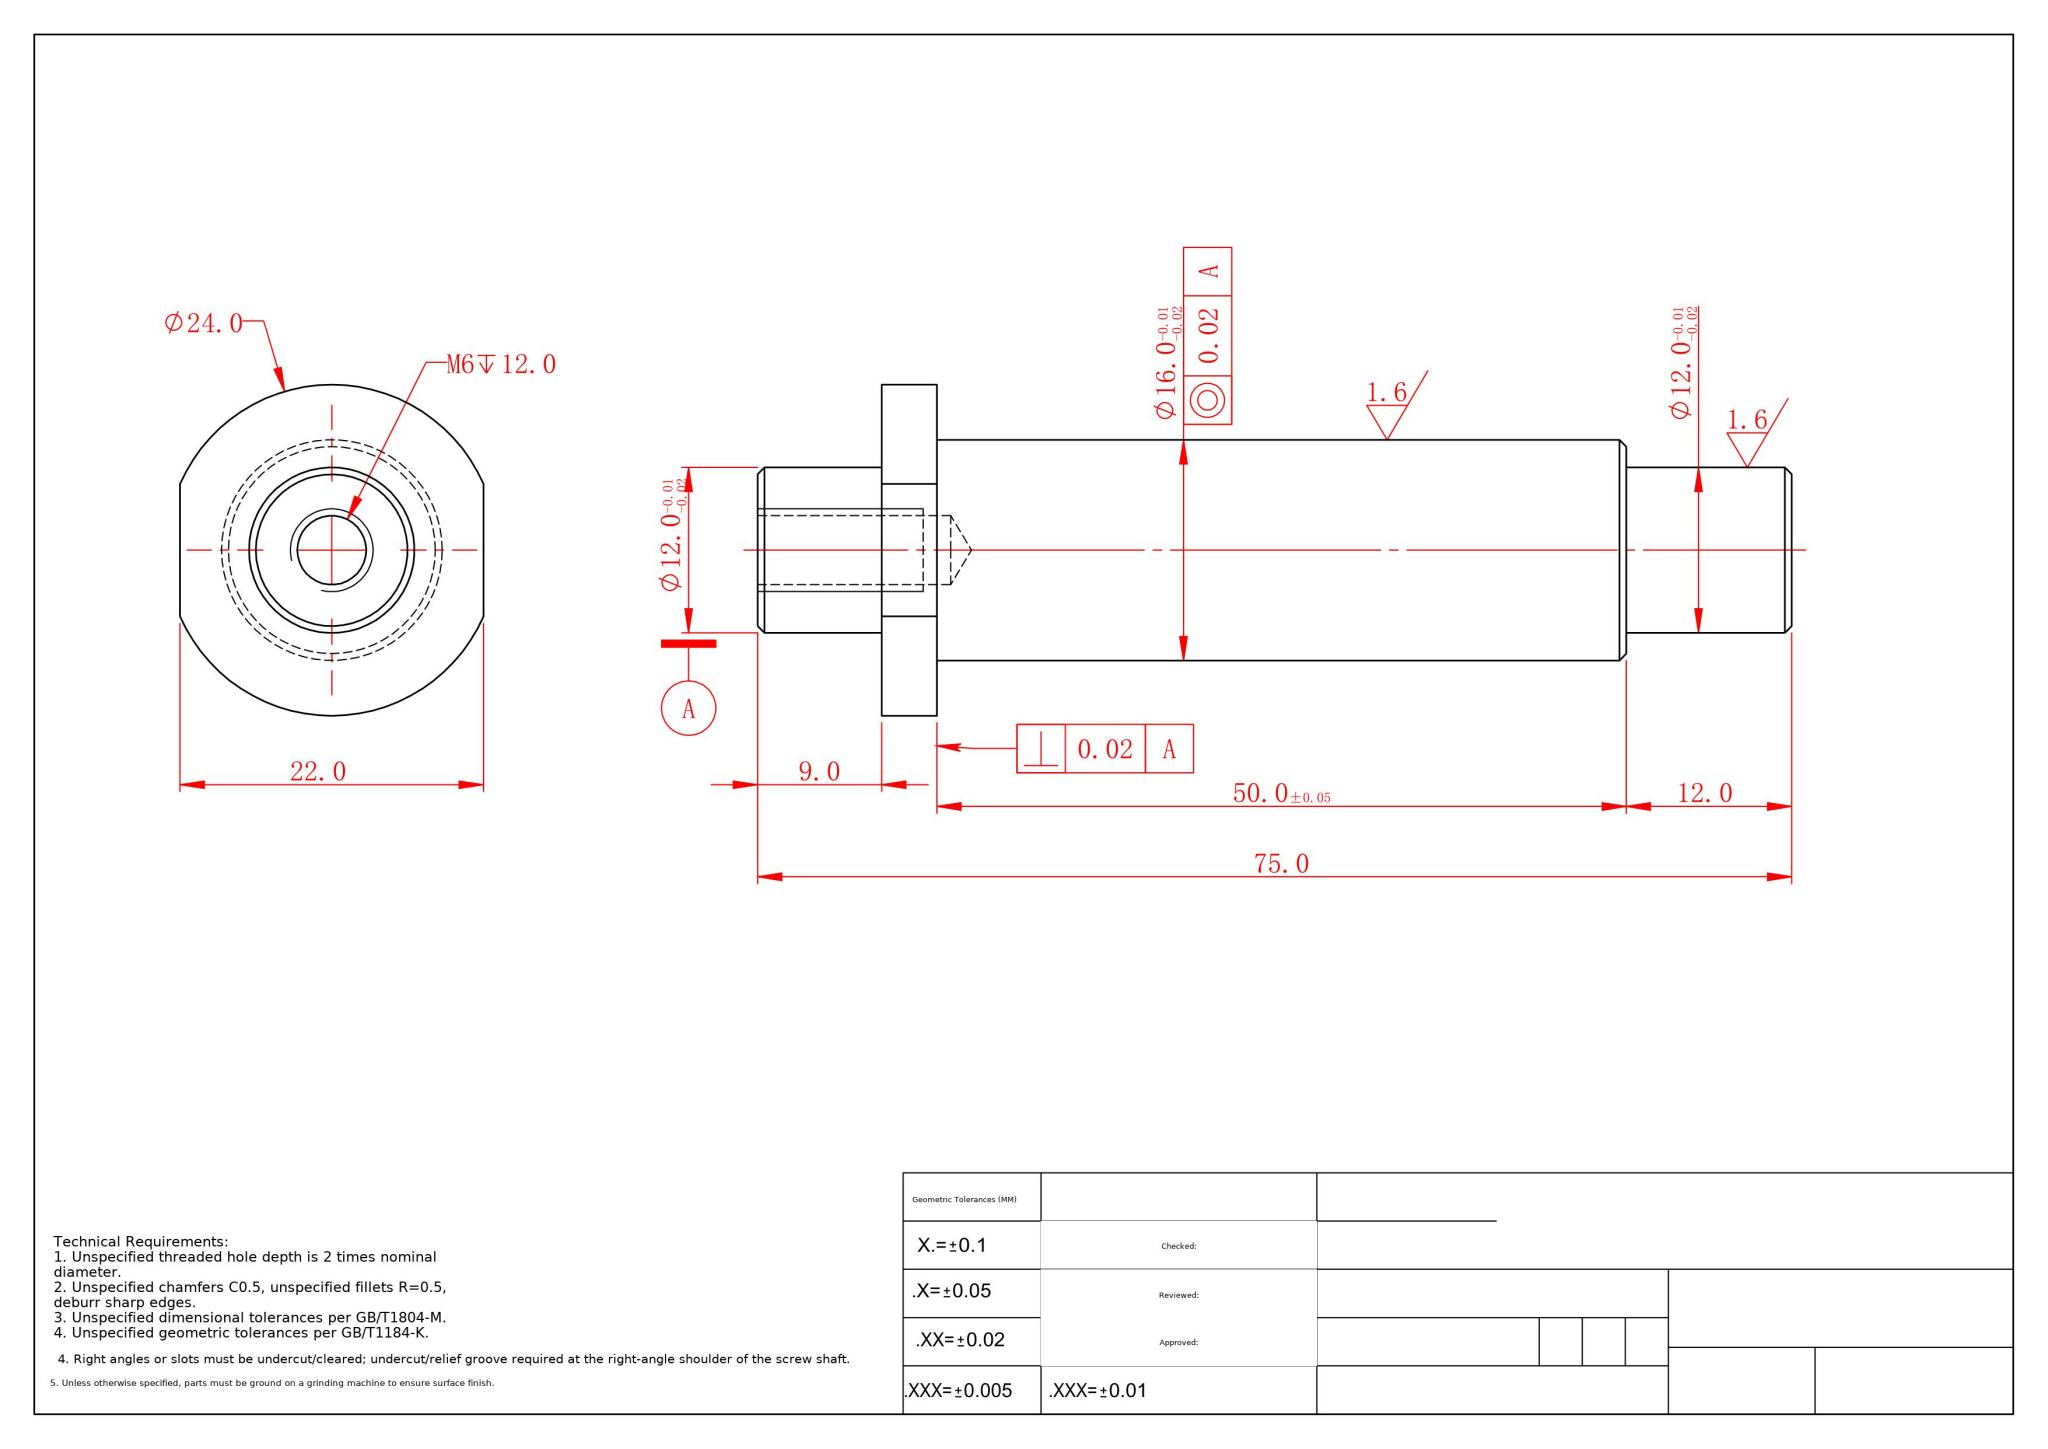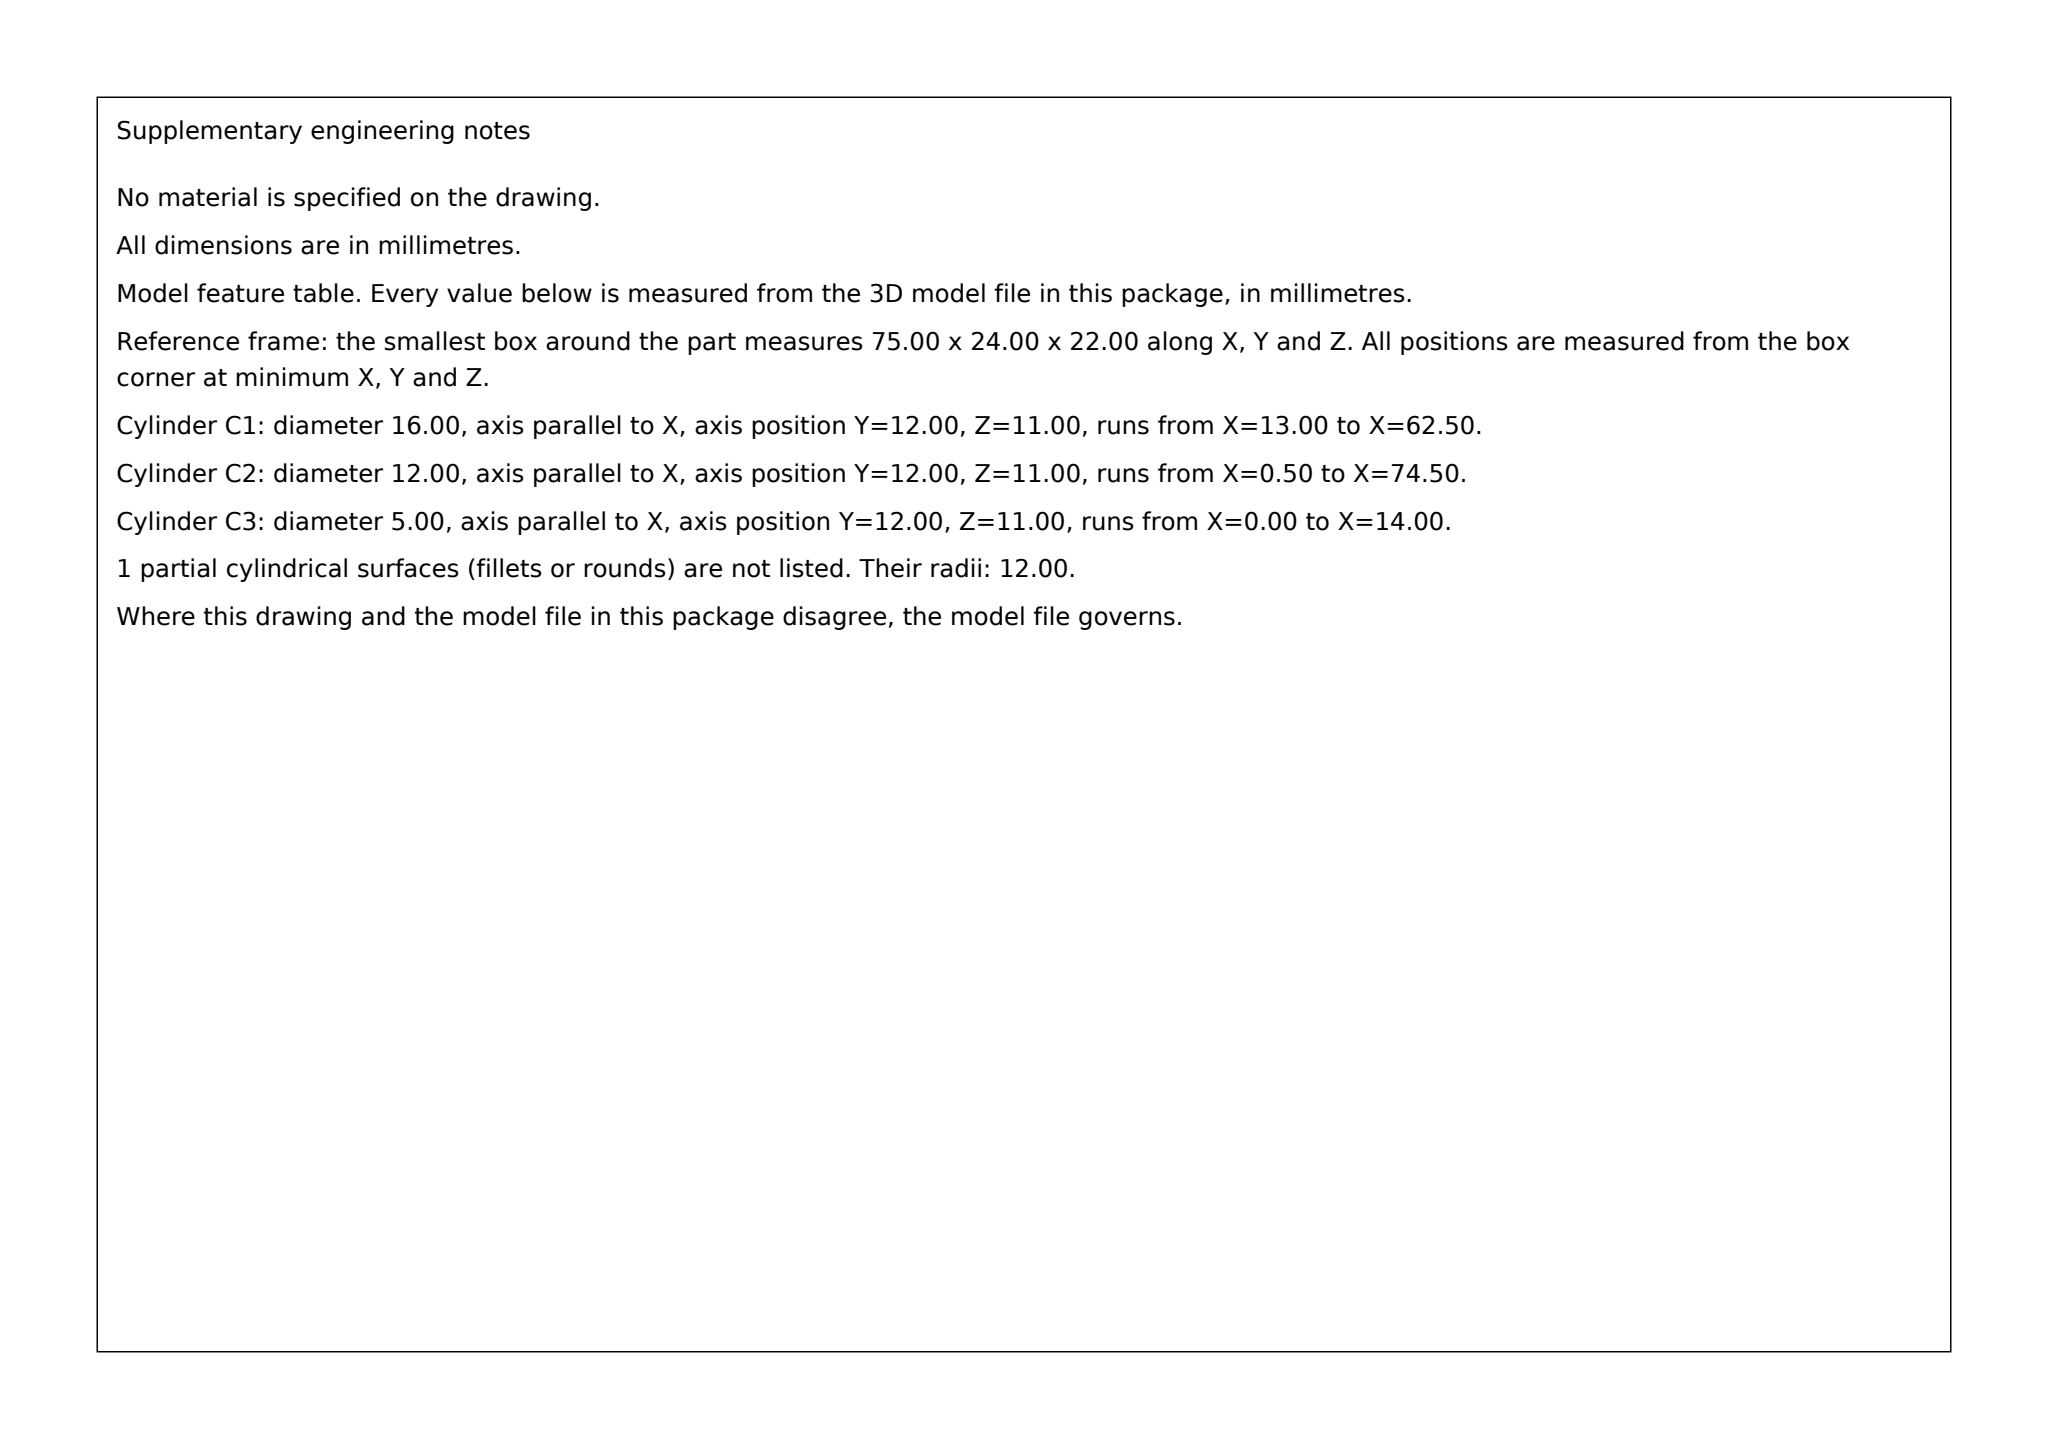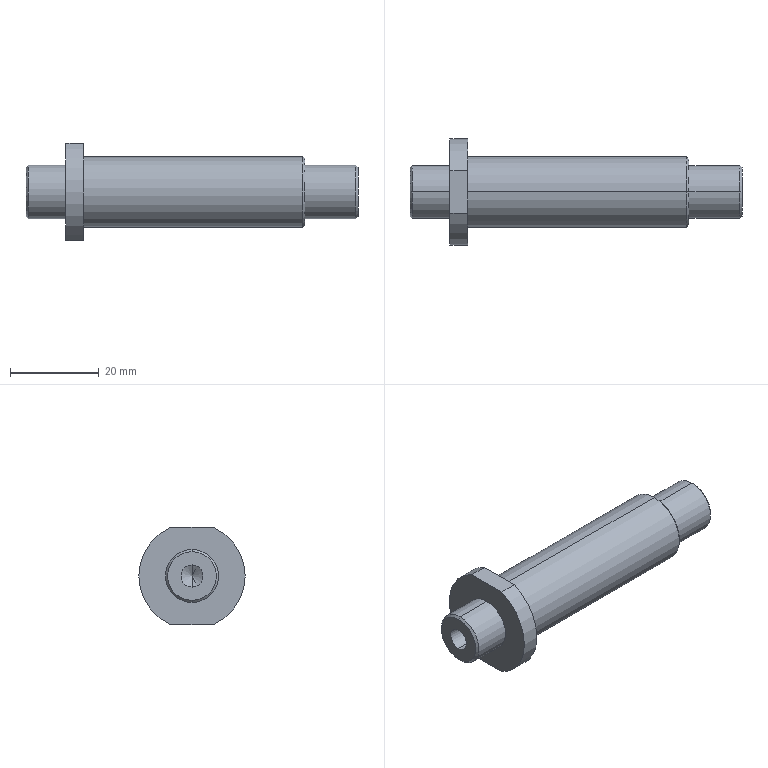Part | SolidWorks | mm | 1 solid | 25 faces | box 75 x 24 x 22 mm | volume 13886 mm3 | cylinder 10 | cone 8 | plane 7 | commonest cylinder face diameters 12 x4 5 x2 16 x2 24 x2
build123d program:
from build123d import *

# Parameters (mm, degrees)
M6_TAPPED_HOLE1_D     = 5
M6_TAPPED_HOLE1_DEPTH = 14
M6_TAPPED_HOLE1_TIP   = 1.502
CUT_EXTRUDE1_REACH    = 66.281
SKETCH4_W             = 1.714
SKETCH4_H             = 24.788
CHAMFER1_SIZE         = 0.5


with BuildPart() as part:
    # Sketch1 → Revolve1 (revolve)
    with BuildSketch(Plane.XY, mode=Mode.PRIVATE) as revolve1_sk:
        Polygon((-37.5, 0), (37.5, 0), (37.5, 6), (25.5, 6), (25.5, 8), (-24.5, 8), (-24.5, 12), (-28.5, 12), (-28.5, 6), (-37.5, 6), align=None)
    revolve(revolve1_sk.sketch.rotate(Axis((0, 0, 0), (1, 0, 0)), 90), axis=Axis((0, 0, 0), (1, 0, 0)))

    # M6 Tapped Hole1
    with Locations(Plane.ZY.offset(37.5)):
        with Locations((0, 0)):
            Hole(M6_TAPPED_HOLE1_D / 2, depth=M6_TAPPED_HOLE1_DEPTH)
            with Locations((0, 0, -(M6_TAPPED_HOLE1_DEPTH + M6_TAPPED_HOLE1_TIP / 2))):  # 118° drill point
                Cone(0, M6_TAPPED_HOLE1_D / 2, M6_TAPPED_HOLE1_TIP, mode=Mode.SUBTRACT)

    # Sketch4 → Cut-Extrude1 (cut, up to next)
    with BuildSketch(Plane(origin=(-24.5, 0, 0), x_dir=(0, 0, -1), z_dir=(1, 0, 0)), mode=Mode.PRIVATE) as cut_extrude1_sk1:
        with Locations((-11.857, 1.847)):
            Rectangle(SKETCH4_W, SKETCH4_H)
    cut_extrude1_tool1 = extrude(cut_extrude1_sk1.sketch, amount=-CUT_EXTRUDE1_REACH, mode=Mode.PRIVATE) & part.part
    # Sketch4 → Cut-Extrude1 (cut, up to next)
    with BuildSketch(Plane(origin=(-24.5, 0, 0), x_dir=(0, 0, -1), z_dir=(1, 0, 0)), mode=Mode.PRIVATE) as cut_extrude1_sk2:
        with Locations((11.857, 1.847)):
            Rectangle(SKETCH4_W, SKETCH4_H)
    cut_extrude1_tool2 = extrude(cut_extrude1_sk2.sketch, amount=-CUT_EXTRUDE1_REACH, mode=Mode.PRIVATE) & part.part
    add(cut_extrude1_tool1.solids().sort_by_distance((-24.5, 1.847, 11.857))[0], mode=Mode.SUBTRACT)
    add(cut_extrude1_tool2.solids().sort_by_distance((-24.5, 1.847, -11.857))[0], mode=Mode.SUBTRACT)

    # Chamfer1
    chamfer1_edges = [part.edges().sort_by_distance(p)[0] for p in [
        (25.5, 0, -8),
        (37.5, 0, -6),
        (-37.5, 0, -6),
    ]]
    chamfer(chamfer1_edges, length=CHAMFER1_SIZE)


solid = part.part
STEP:
#1=CARTESIAN_POINT('',(37.5,0.,-5.5));
#2=VERTEX_POINT('',#1);
#3=CARTESIAN_POINT('',(37.5,0.,5.5));
#4=VERTEX_POINT('',#3);
#5=CARTESIAN_POINT('',(37.5,0.,0.));
#6=DIRECTION('',(1.,0.,0.));
#7=DIRECTION('',(0.,0.,1.));
#8=AXIS2_PLACEMENT_3D('',#5,#6,#7);
#9=CIRCLE('',#8,5.5);
#10=EDGE_CURVE('',#2,#4,#9,.T.);
#11=ORIENTED_EDGE('',*,*,#10,.F.);
#12=CARTESIAN_POINT('',(37.,0.,-6.));
#13=VERTEX_POINT('',#12);
#14=CARTESIAN_POINT('',(37.,0.,-6.));
#15=DIRECTION('',(-0.7071,0.,-0.7071));
#16=VECTOR('',#15,1000.);
#17=LINE('',#14,#16);
#18=EDGE_CURVE('',#2,#13,#17,.T.);
#19=ORIENTED_EDGE('',*,*,#18,.T.);
#20=CARTESIAN_POINT('',(37.,0.,6.));
#21=VERTEX_POINT('',#20);
#22=CARTESIAN_POINT('',(37.,0.,0.));
#23=DIRECTION('',(-1.,0.,0.));
#24=DIRECTION('',(0.,0.,1.));
#25=AXIS2_PLACEMENT_3D('',#22,#23,#24);
#26=CIRCLE('',#25,6.);
#27=EDGE_CURVE('',#21,#13,#26,.T.);
#28=ORIENTED_EDGE('',*,*,#27,.F.);
#29=CARTESIAN_POINT('',(37.,0.,6.));
#30=DIRECTION('',(-0.7071,0.,0.7071));
#31=VECTOR('',#30,1000.);
#32=LINE('',#29,#31);
#33=EDGE_CURVE('',#4,#21,#32,.T.);
#34=ORIENTED_EDGE('',*,*,#33,.F.);
#35=EDGE_LOOP('',(#11,#19,#28,#34));
#36=FACE_OUTER_BOUND('',#35,.T.);
#37=CARTESIAN_POINT('',(37.,0.,0.));
#38=DIRECTION('',(-1.,0.,0.));
#39=DIRECTION('',(0.,0.,1.));
#40=AXIS2_PLACEMENT_3D('',#37,#38,#39);
#41=CONICAL_SURFACE('',#40,6.,0.7854);
#42=ADVANCED_FACE('',(#36),#41,.T.);
#43=CARTESIAN_POINT('',(25.5,0.,-7.5));
#44=VERTEX_POINT('',#43);
#45=CARTESIAN_POINT('',(25.5,0.,7.5));
#46=VERTEX_POINT('',#45);
#47=CARTESIAN_POINT('',(25.5,0.,0.));
#48=DIRECTION('',(1.,0.,0.));
#49=DIRECTION('',(0.,0.,1.));
#50=AXIS2_PLACEMENT_3D('',#47,#48,#49);
#51=CIRCLE('',#50,7.5);
#52=EDGE_CURVE('',#44,#46,#51,.T.);
#53=ORIENTED_EDGE('',*,*,#52,.F.);
#54=CARTESIAN_POINT('',(25.,0.,-8.));
#55=VERTEX_POINT('',#54);
#56=CARTESIAN_POINT('',(25.,0.,-8.));
#57=DIRECTION('',(-0.7071,0.,-0.7071));
#58=VECTOR('',#57,1000.);
#59=LINE('',#56,#58);
#60=EDGE_CURVE('',#44,#55,#59,.T.);
#61=ORIENTED_EDGE('',*,*,#60,.T.);
#62=CARTESIAN_POINT('',(25.,0.,8.));
#63=VERTEX_POINT('',#62);
#64=CARTESIAN_POINT('',(25.,0.,0.));
#65=DIRECTION('',(-1.,0.,0.));
#66=DIRECTION('',(0.,0.,1.));
#67=AXIS2_PLACEMENT_3D('',#64,#65,#66);
#68=CIRCLE('',#67,8.);
#69=EDGE_CURVE('',#63,#55,#68,.T.);
#70=ORIENTED_EDGE('',*,*,#69,.F.);
#71=CARTESIAN_POINT('',(25.,0.,8.));
#72=DIRECTION('',(-0.7071,0.,0.7071));
#73=VECTOR('',#72,1000.);
#74=LINE('',#71,#73);
#75=EDGE_CURVE('',#46,#63,#74,.T.);
#76=ORIENTED_EDGE('',*,*,#75,.F.);
#77=EDGE_LOOP('',(#53,#61,#70,#76));
#78=FACE_OUTER_BOUND('',#77,.T.);
#79=CARTESIAN_POINT('',(25.,0.,0.));
#80=DIRECTION('',(-1.,0.,0.));
#81=DIRECTION('',(0.,0.,1.));
#82=AXIS2_PLACEMENT_3D('',#79,#80,#81);
#83=CONICAL_SURFACE('',#82,8.,0.7854);
#84=ADVANCED_FACE('',(#78),#83,.T.);
#85=CARTESIAN_POINT('',(-37.5,0.,5.5));
#86=VERTEX_POINT('',#85);
#87=CARTESIAN_POINT('',(-37.5,0.,-5.5));
#88=VERTEX_POINT('',#87);
#89=CARTESIAN_POINT('',(-37.5,0.,0.));
#90=DIRECTION('',(-1.,0.,0.));
#91=DIRECTION('',(0.,0.,-1.));
#92=AXIS2_PLACEMENT_3D('',#89,#90,#91);
#93=CIRCLE('',#92,5.5);
#94=EDGE_CURVE('',#86,#88,#93,.T.);
#95=ORIENTED_EDGE('',*,*,#94,.F.);
#96=CARTESIAN_POINT('',(-37.,0.,6.));
#97=VERTEX_POINT('',#96);
#98=CARTESIAN_POINT('',(-37.5,0.,5.5));
#99=DIRECTION('',(0.7071,0.,0.7071));
#100=VECTOR('',#99,1000.);
#101=LINE('',#98,#100);
#102=EDGE_CURVE('',#86,#97,#101,.T.);
#103=ORIENTED_EDGE('',*,*,#102,.T.);
#104=CARTESIAN_POINT('',(-37.,0.,-6.));
#105=VERTEX_POINT('',#104);
#106=CARTESIAN_POINT('',(-37.,0.,0.));
#107=DIRECTION('',(1.,0.,0.));
#108=DIRECTION('',(0.,0.,-1.));
#109=AXIS2_PLACEMENT_3D('',#106,#107,#108);
#110=CIRCLE('',#109,6.);
#111=EDGE_CURVE('',#105,#97,#110,.T.);
#112=ORIENTED_EDGE('',*,*,#111,.F.);
#113=CARTESIAN_POINT('',(-37.5,0.,-5.5));
#114=DIRECTION('',(0.7071,0.,-0.7071));
#115=VECTOR('',#114,1000.);
#116=LINE('',#113,#115);
#117=EDGE_CURVE('',#88,#105,#116,.T.);
#118=ORIENTED_EDGE('',*,*,#117,.F.);
#119=EDGE_LOOP('',(#95,#103,#112,#118));
#120=FACE_OUTER_BOUND('',#119,.T.);
#121=CARTESIAN_POINT('',(-37.5,0.,0.));
#122=DIRECTION('',(1.,0.,0.));
#123=DIRECTION('',(0.,0.,-1.));
#124=AXIS2_PLACEMENT_3D('',#121,#122,#123);
#125=CONICAL_SURFACE('',#124,5.5,0.7854);
#126=ADVANCED_FACE('',(#120),#125,.T.);
#127=CARTESIAN_POINT('',(-23.5,0.,-2.5));
#128=VERTEX_POINT('',#127);
#129=CARTESIAN_POINT('',(-23.5,0.,2.5));
#130=VERTEX_POINT('',#129);
#131=CARTESIAN_POINT('',(-23.5,0.,0.));
#132=DIRECTION('',(-1.,0.,0.));
#133=DIRECTION('',(0.,0.,1.));
#134=AXIS2_PLACEMENT_3D('',#131,#132,#133);
#135=CIRCLE('',#134,2.5);
#136=EDGE_CURVE('',#128,#130,#135,.T.);
#137=ORIENTED_EDGE('',*,*,#136,.F.);
#138=CARTESIAN_POINT('',(-37.5,0.,-2.5));
#139=VERTEX_POINT('',#138);
#140=CARTESIAN_POINT('',(-37.5,0.,-2.5));
#141=DIRECTION('',(-1.,0.,0.));
#142=VECTOR('',#141,1000.);
#143=LINE('',#140,#142);
#144=EDGE_CURVE('',#128,#139,#143,.T.);
#145=ORIENTED_EDGE('',*,*,#144,.T.);
#146=CARTESIAN_POINT('',(-37.5,0.,2.5));
#147=VERTEX_POINT('',#146);
#148=CARTESIAN_POINT('',(-37.5,0.,0.));
#149=DIRECTION('',(-1.,0.,0.));
#150=DIRECTION('',(0.,0.,1.));
#151=AXIS2_PLACEMENT_3D('',#148,#149,#150);
#152=CIRCLE('',#151,2.5);
#153=EDGE_CURVE('',#139,#147,#152,.T.);
#154=ORIENTED_EDGE('',*,*,#153,.T.);
#155=CARTESIAN_POINT('',(-37.5,0.,2.5));
#156=DIRECTION('',(-1.,0.,0.));
#157=VECTOR('',#156,1000.);
#158=LINE('',#155,#157);
#159=EDGE_CURVE('',#130,#147,#158,.T.);
#160=ORIENTED_EDGE('',*,*,#159,.F.);
#161=EDGE_LOOP('',(#137,#145,#154,#160));
#162=FACE_OUTER_BOUND('',#161,.T.);
#163=CARTESIAN_POINT('',(-37.5,0.,0.));
#164=DIRECTION('',(-1.,0.,0.));
#165=DIRECTION('',(0.,0.,1.));
#166=AXIS2_PLACEMENT_3D('',#163,#164,#165);
#167=CYLINDRICAL_SURFACE('',#166,2.5);
#168=ADVANCED_FACE('',(#162),#167,.F.);
#169=CARTESIAN_POINT('',(-21.998,-0.,0.));
#170=VERTEX_POINT('',#169);
#171=CARTESIAN_POINT('',(-23.5,0.,2.5));
#172=DIRECTION('',(-0.515,0.,0.8572));
#173=VECTOR('',#172,1000.);
#174=LINE('',#171,#173);
#175=EDGE_CURVE('',#170,#130,#174,.T.);
#176=ORIENTED_EDGE('',*,*,#175,.F.);
#177=CARTESIAN_POINT('',(-23.5,0.,-2.5));
#178=DIRECTION('',(-0.515,0.,-0.8572));
#179=VECTOR('',#178,1000.);
#180=LINE('',#177,#179);
#181=EDGE_CURVE('',#170,#128,#180,.T.);
#182=ORIENTED_EDGE('',*,*,#181,.T.);
#183=ORIENTED_EDGE('',*,*,#136,.T.);
#184=EDGE_LOOP('',(#176,#182,#183));
#185=FACE_OUTER_BOUND('',#184,.T.);
#186=CARTESIAN_POINT('',(-23.5,0.,0.));
#187=DIRECTION('',(-1.,0.,0.));
#188=DIRECTION('',(0.,0.,1.));
#189=AXIS2_PLACEMENT_3D('',#186,#187,#188);
#190=CONICAL_SURFACE('',#189,2.5,1.03);
#191=ADVANCED_FACE('',(#185),#190,.F.);
#192=CARTESIAN_POINT('',(-28.5,0.,6.));
#193=VERTEX_POINT('',#192);
#194=CARTESIAN_POINT('',(-28.5,0.,-6.));
#195=VERTEX_POINT('',#194);
#196=CARTESIAN_POINT('',(-28.5,0.,0.));
#197=DIRECTION('',(-1.,0.,0.));
#198=DIRECTION('',(0.,0.,1.));
#199=AXIS2_PLACEMENT_3D('',#196,#197,#198);
#200=CIRCLE('',#199,6.);
#201=EDGE_CURVE('',#193,#195,#200,.T.);
#202=ORIENTED_EDGE('',*,*,#201,.T.);
#203=CARTESIAN_POINT('',(0.,0.,-6.));
#204=DIRECTION('',(-1.,0.,0.));
#205=VECTOR('',#204,1000.);
#206=LINE('',#203,#205);
#207=EDGE_CURVE('',#195,#105,#206,.T.);
#208=ORIENTED_EDGE('',*,*,#207,.T.);
#209=ORIENTED_EDGE('',*,*,#111,.T.);
#210=CARTESIAN_POINT('',(0.,0.,6.));
#211=DIRECTION('',(-1.,0.,0.));
#212=VECTOR('',#211,1000.);
#213=LINE('',#210,#212);
#214=EDGE_CURVE('',#193,#97,#213,.T.);
#215=ORIENTED_EDGE('',*,*,#214,.F.);
#216=EDGE_LOOP('',(#202,#208,#209,#215));
#217=FACE_OUTER_BOUND('',#216,.T.);
#218=CARTESIAN_POINT('',(0.,0.,0.));
#219=DIRECTION('',(-1.,0.,0.));
#220=DIRECTION('',(0.,0.,1.));
#221=AXIS2_PLACEMENT_3D('',#218,#219,#220);
#222=CYLINDRICAL_SURFACE('',#221,6.);
#223=ADVANCED_FACE('',(#217),#222,.T.);
#224=ORIENTED_EDGE('',*,*,#69,.T.);
#225=CARTESIAN_POINT('',(-24.5,0.,-8.));
#226=VERTEX_POINT('',#225);
#227=CARTESIAN_POINT('',(0.,0.,-8.));
#228=DIRECTION('',(-1.,0.,0.));
#229=VECTOR('',#228,1000.);
#230=LINE('',#227,#229);
#231=EDGE_CURVE('',#55,#226,#230,.T.);
#232=ORIENTED_EDGE('',*,*,#231,.T.);
#233=CARTESIAN_POINT('',(-24.5,0.,8.));
#234=VERTEX_POINT('',#233);
#235=CARTESIAN_POINT('',(-24.5,0.,0.));
#236=DIRECTION('',(-1.,0.,0.));
#237=DIRECTION('',(0.,0.,1.));
#238=AXIS2_PLACEMENT_3D('',#235,#236,#237);
#239=CIRCLE('',#238,8.);
#240=EDGE_CURVE('',#234,#226,#239,.T.);
#241=ORIENTED_EDGE('',*,*,#240,.F.);
#242=CARTESIAN_POINT('',(0.,0.,8.));
#243=DIRECTION('',(-1.,0.,0.));
#244=VECTOR('',#243,1000.);
#245=LINE('',#242,#244);
#246=EDGE_CURVE('',#63,#234,#245,.T.);
#247=ORIENTED_EDGE('',*,*,#246,.F.);
#248=EDGE_LOOP('',(#224,#232,#241,#247));
#249=FACE_OUTER_BOUND('',#248,.T.);
#250=CARTESIAN_POINT('',(0.,0.,0.));
#251=DIRECTION('',(-1.,0.,0.));
#252=DIRECTION('',(0.,0.,1.));
#253=AXIS2_PLACEMENT_3D('',#250,#251,#252);
#254=CYLINDRICAL_SURFACE('',#253,8.);
#255=ADVANCED_FACE('',(#249),#254,.T.);
#256=ORIENTED_EDGE('',*,*,#27,.T.);
#257=CARTESIAN_POINT('',(25.5,0.,-6.));
#258=VERTEX_POINT('',#257);
#259=CARTESIAN_POINT('',(0.,0.,-6.));
#260=DIRECTION('',(-1.,0.,0.));
#261=VECTOR('',#260,1000.);
#262=LINE('',#259,#261);
#263=EDGE_CURVE('',#13,#258,#262,.T.);
#264=ORIENTED_EDGE('',*,*,#263,.T.);
#265=CARTESIAN_POINT('',(25.5,0.,6.));
#266=VERTEX_POINT('',#265);
#267=CARTESIAN_POINT('',(25.5,0.,0.));
#268=DIRECTION('',(-1.,0.,0.));
#269=DIRECTION('',(0.,0.,1.));
#270=AXIS2_PLACEMENT_3D('',#267,#268,#269);
#271=CIRCLE('',#270,6.);
#272=EDGE_CURVE('',#266,#258,#271,.T.);
#273=ORIENTED_EDGE('',*,*,#272,.F.);
#274=CARTESIAN_POINT('',(0.,0.,6.));
#275=DIRECTION('',(-1.,0.,0.));
#276=VECTOR('',#275,1000.);
#277=LINE('',#274,#276);
#278=EDGE_CURVE('',#21,#266,#277,.T.);
#279=ORIENTED_EDGE('',*,*,#278,.F.);
#280=EDGE_LOOP('',(#256,#264,#273,#279));
#281=FACE_OUTER_BOUND('',#280,.T.);
#282=CARTESIAN_POINT('',(0.,0.,0.));
#283=DIRECTION('',(-1.,0.,0.));
#284=DIRECTION('',(0.,0.,1.));
#285=AXIS2_PLACEMENT_3D('',#282,#283,#284);
#286=CYLINDRICAL_SURFACE('',#285,6.);
#287=ADVANCED_FACE('',(#281),#286,.T.);
#288=CARTESIAN_POINT('',(-24.5,4.796,11.));
#289=VERTEX_POINT('',#288);
#290=CARTESIAN_POINT('',(-24.5,4.796,-11.));
#291=VERTEX_POINT('',#290);
#292=CARTESIAN_POINT('',(-24.5,0.,0.));
#293=DIRECTION('',(-1.,0.,0.));
#294=DIRECTION('',(0.,0.,1.));
#295=AXIS2_PLACEMENT_3D('',#292,#293,#294);
#296=CIRCLE('',#295,12.);
#297=EDGE_CURVE('',#289,#291,#296,.T.);
#298=ORIENTED_EDGE('',*,*,#297,.T.);
#299=CARTESIAN_POINT('',(-28.5,4.796,-11.));
#300=VERTEX_POINT('',#299);
#301=CARTESIAN_POINT('',(0.,4.796,-11.));
#302=DIRECTION('',(1.,0.,0.));
#303=VECTOR('',#302,1000.);
#304=LINE('',#301,#303);
#305=EDGE_CURVE('',#300,#291,#304,.T.);
#306=ORIENTED_EDGE('',*,*,#305,.F.);
#307=CARTESIAN_POINT('',(-28.5,4.796,11.));
#308=VERTEX_POINT('',#307);
#309=CARTESIAN_POINT('',(-28.5,0.,0.));
#310=DIRECTION('',(-1.,0.,0.));
#311=DIRECTION('',(0.,0.,1.));
#312=AXIS2_PLACEMENT_3D('',#309,#310,#311);
#313=CIRCLE('',#312,12.);
#314=EDGE_CURVE('',#308,#300,#313,.T.);
#315=ORIENTED_EDGE('',*,*,#314,.F.);
#316=CARTESIAN_POINT('',(0.,4.796,11.));
#317=DIRECTION('',(-1.,0.,0.));
#318=VECTOR('',#317,1000.);
#319=LINE('',#316,#318);
#320=EDGE_CURVE('',#289,#308,#319,.T.);
#321=ORIENTED_EDGE('',*,*,#320,.F.);
#322=EDGE_LOOP('',(#298,#306,#315,#321));
#323=FACE_OUTER_BOUND('',#322,.T.);
#324=CARTESIAN_POINT('',(0.,0.,0.));
#325=DIRECTION('',(-1.,0.,0.));
#326=DIRECTION('',(0.,0.,1.));
#327=AXIS2_PLACEMENT_3D('',#324,#325,#326);
#328=CYLINDRICAL_SURFACE('',#327,12.);
#329=ADVANCED_FACE('',(#323),#328,.T.);
#330=CARTESIAN_POINT('',(37.5,0.,0.));
#331=DIRECTION('',(1.,0.,0.));
#332=DIRECTION('',(0.,0.,1.));
#333=AXIS2_PLACEMENT_3D('',#330,#331,#332);
#334=CIRCLE('',#333,5.5);
#335=EDGE_CURVE('',#4,#2,#334,.T.);
#336=ORIENTED_EDGE('',*,*,#335,.T.);
#337=ORIENTED_EDGE('',*,*,#10,.T.);
#338=EDGE_LOOP('',(#336,#337));
#339=FACE_OUTER_BOUND('',#338,.T.);
#340=CARTESIAN_POINT('',(37.5,0.,0.));
#341=DIRECTION('',(-1.,0.,0.));
#342=DIRECTION('',(0.,0.,1.));
#343=AXIS2_PLACEMENT_3D('',#340,#341,#342);
#344=PLANE('',#343);
#345=ADVANCED_FACE('',(#339),#344,.F.);
#346=ORIENTED_EDGE('',*,*,#263,.F.);
#347=CARTESIAN_POINT('',(37.,0.,0.));
#348=DIRECTION('',(-1.,0.,0.));
#349=DIRECTION('',(0.,0.,1.));
#350=AXIS2_PLACEMENT_3D('',#347,#348,#349);
#351=CIRCLE('',#350,6.);
#352=EDGE_CURVE('',#13,#21,#351,.T.);
#353=ORIENTED_EDGE('',*,*,#352,.T.);
#354=ORIENTED_EDGE('',*,*,#278,.T.);
#355=CARTESIAN_POINT('',(25.5,0.,0.));
#356=DIRECTION('',(-1.,0.,0.));
#357=DIRECTION('',(0.,0.,1.));
#358=AXIS2_PLACEMENT_3D('',#355,#356,#357);
#359=CIRCLE('',#358,6.);
#360=EDGE_CURVE('',#258,#266,#359,.T.);
#361=ORIENTED_EDGE('',*,*,#360,.F.);
#362=EDGE_LOOP('',(#346,#353,#354,#361));
#363=FACE_OUTER_BOUND('',#362,.T.);
#364=CARTESIAN_POINT('',(0.,0.,0.));
#365=DIRECTION('',(-1.,0.,0.));
#366=DIRECTION('',(0.,0.,1.));
#367=AXIS2_PLACEMENT_3D('',#364,#365,#366);
#368=CYLINDRICAL_SURFACE('',#367,6.);
#369=ADVANCED_FACE('',(#363),#368,.T.);
#370=CARTESIAN_POINT('',(25.5,0.,0.));
#371=DIRECTION('',(1.,0.,0.));
#372=DIRECTION('',(0.,0.,1.));
#373=AXIS2_PLACEMENT_3D('',#370,#371,#372);
#374=CIRCLE('',#373,7.5);
#375=EDGE_CURVE('',#46,#44,#374,.T.);
#376=ORIENTED_EDGE('',*,*,#375,.T.);
#377=ORIENTED_EDGE('',*,*,#52,.T.);
#378=EDGE_LOOP('',(#376,#377));
#379=FACE_OUTER_BOUND('',#378,.T.);
#380=ORIENTED_EDGE('',*,*,#272,.T.);
#381=ORIENTED_EDGE('',*,*,#360,.T.);
#382=EDGE_LOOP('',(#380,#381));
#383=FACE_BOUND('',#382,.T.);
#384=CARTESIAN_POINT('',(25.5,6.,0.));
#385=DIRECTION('',(-1.,0.,0.));
#386=DIRECTION('',(0.,0.,1.));
#387=AXIS2_PLACEMENT_3D('',#384,#385,#386);
#388=PLANE('',#387);
#389=ADVANCED_FACE('',(#379,#383),#388,.F.);
#390=ORIENTED_EDGE('',*,*,#231,.F.);
#391=CARTESIAN_POINT('',(25.,0.,0.));
#392=DIRECTION('',(-1.,0.,0.));
#393=DIRECTION('',(0.,0.,1.));
#394=AXIS2_PLACEMENT_3D('',#391,#392,#393);
#395=CIRCLE('',#394,8.);
#396=EDGE_CURVE('',#55,#63,#395,.T.);
#397=ORIENTED_EDGE('',*,*,#396,.T.);
#398=ORIENTED_EDGE('',*,*,#246,.T.);
#399=CARTESIAN_POINT('',(-24.5,0.,0.));
#400=DIRECTION('',(-1.,0.,0.));
#401=DIRECTION('',(0.,0.,1.));
#402=AXIS2_PLACEMENT_3D('',#399,#400,#401);
#403=CIRCLE('',#402,8.);
#404=EDGE_CURVE('',#226,#234,#403,.T.);
#405=ORIENTED_EDGE('',*,*,#404,.F.);
#406=EDGE_LOOP('',(#390,#397,#398,#405));
#407=FACE_OUTER_BOUND('',#406,.T.);
#408=CARTESIAN_POINT('',(0.,0.,0.));
#409=DIRECTION('',(-1.,0.,0.));
#410=DIRECTION('',(0.,0.,1.));
#411=AXIS2_PLACEMENT_3D('',#408,#409,#410);
#412=CYLINDRICAL_SURFACE('',#411,8.);
#413=ADVANCED_FACE('',(#407),#412,.T.);
#414=CARTESIAN_POINT('',(-24.5,-4.796,-11.));
#415=VERTEX_POINT('',#414);
#416=CARTESIAN_POINT('',(-24.5,-4.796,11.));
#417=VERTEX_POINT('',#416);
#418=CARTESIAN_POINT('',(-24.5,0.,0.));
#419=DIRECTION('',(-1.,0.,0.));
#420=DIRECTION('',(0.,0.,1.));
#421=AXIS2_PLACEMENT_3D('',#418,#419,#420);
#422=CIRCLE('',#421,12.);
#423=EDGE_CURVE('',#415,#417,#422,.T.);
#424=ORIENTED_EDGE('',*,*,#423,.F.);
#425=CARTESIAN_POINT('',(-24.5,14.241,-11.));
#426=DIRECTION('',(0.,-1.,0.));
#427=VECTOR('',#426,1000.);
#428=LINE('',#425,#427);
#429=EDGE_CURVE('',#291,#415,#428,.T.);
#430=ORIENTED_EDGE('',*,*,#429,.F.);
#431=ORIENTED_EDGE('',*,*,#297,.F.);
#432=CARTESIAN_POINT('',(-24.5,14.241,11.));
#433=DIRECTION('',(0.,1.,0.));
#434=VECTOR('',#433,1000.);
#435=LINE('',#432,#434);
#436=EDGE_CURVE('',#417,#289,#435,.T.);
#437=ORIENTED_EDGE('',*,*,#436,.F.);
#438=EDGE_LOOP('',(#424,#430,#431,#437));
#439=FACE_OUTER_BOUND('',#438,.T.);
#440=ORIENTED_EDGE('',*,*,#240,.T.);
#441=ORIENTED_EDGE('',*,*,#404,.T.);
#442=EDGE_LOOP('',(#440,#441));
#443=FACE_BOUND('',#442,.T.);
#444=CARTESIAN_POINT('',(-24.5,8.,0.));
#445=DIRECTION('',(-1.,0.,0.));
#446=DIRECTION('',(0.,0.,1.));
#447=AXIS2_PLACEMENT_3D('',#444,#445,#446);
#448=PLANE('',#447);
#449=ADVANCED_FACE('',(#439,#443),#448,.F.);
#450=CARTESIAN_POINT('',(-28.5,-4.796,-11.));
#451=VERTEX_POINT('',#450);
#452=CARTESIAN_POINT('',(-28.5,-4.796,11.));
#453=VERTEX_POINT('',#452);
#454=CARTESIAN_POINT('',(-28.5,0.,0.));
#455=DIRECTION('',(-1.,0.,0.));
#456=DIRECTION('',(0.,0.,1.));
#457=AXIS2_PLACEMENT_3D('',#454,#455,#456);
#458=CIRCLE('',#457,12.);
#459=EDGE_CURVE('',#451,#453,#458,.T.);
#460=ORIENTED_EDGE('',*,*,#459,.F.);
#461=CARTESIAN_POINT('',(0.,-4.796,-11.));
#462=DIRECTION('',(-1.,0.,0.));
#463=VECTOR('',#462,1000.);
#464=LINE('',#461,#463);
#465=EDGE_CURVE('',#415,#451,#464,.T.);
#466=ORIENTED_EDGE('',*,*,#465,.F.);
#467=ORIENTED_EDGE('',*,*,#423,.T.);
#468=CARTESIAN_POINT('',(0.,-4.796,11.));
#469=DIRECTION('',(1.,0.,0.));
#470=VECTOR('',#469,1000.);
#471=LINE('',#468,#470);
#472=EDGE_CURVE('',#453,#417,#471,.T.);
#473=ORIENTED_EDGE('',*,*,#472,.F.);
#474=EDGE_LOOP('',(#460,#466,#467,#473));
#475=FACE_OUTER_BOUND('',#474,.T.);
#476=CARTESIAN_POINT('',(0.,0.,0.));
#477=DIRECTION('',(-1.,0.,0.));
#478=DIRECTION('',(0.,0.,1.));
#479=AXIS2_PLACEMENT_3D('',#476,#477,#478);
#480=CYLINDRICAL_SURFACE('',#479,12.);
#481=ADVANCED_FACE('',(#475),#480,.T.);
#482=ORIENTED_EDGE('',*,*,#201,.F.);
#483=CARTESIAN_POINT('',(-28.5,0.,0.));
#484=DIRECTION('',(-1.,0.,0.));
#485=DIRECTION('',(0.,0.,1.));
#486=AXIS2_PLACEMENT_3D('',#483,#484,#485);
#487=CIRCLE('',#486,6.);
#488=EDGE_CURVE('',#195,#193,#487,.T.);
#489=ORIENTED_EDGE('',*,*,#488,.F.);
#490=EDGE_LOOP('',(#482,#489));
#491=FACE_BOUND('',#490,.T.);
#492=ORIENTED_EDGE('',*,*,#314,.T.);
#493=CARTESIAN_POINT('',(-28.5,14.241,-11.));
#494=DIRECTION('',(0.,1.,0.));
#495=VECTOR('',#494,1000.);
#496=LINE('',#493,#495);
#497=EDGE_CURVE('',#451,#300,#496,.T.);
#498=ORIENTED_EDGE('',*,*,#497,.F.);
#499=ORIENTED_EDGE('',*,*,#459,.T.);
#500=CARTESIAN_POINT('',(-28.5,14.241,11.));
#501=DIRECTION('',(0.,-1.,0.));
#502=VECTOR('',#501,1000.);
#503=LINE('',#500,#502);
#504=EDGE_CURVE('',#308,#453,#503,.T.);
#505=ORIENTED_EDGE('',*,*,#504,.F.);
#506=EDGE_LOOP('',(#492,#498,#499,#505));
#507=FACE_OUTER_BOUND('',#506,.T.);
#508=CARTESIAN_POINT('',(-28.5,12.,0.));
#509=DIRECTION('',(1.,0.,0.));
#510=DIRECTION('',(0.,0.,-1.));
#511=AXIS2_PLACEMENT_3D('',#508,#509,#510);
#512=PLANE('',#511);
#513=ADVANCED_FACE('',(#491,#507),#512,.F.);
#514=ORIENTED_EDGE('',*,*,#207,.F.);
#515=ORIENTED_EDGE('',*,*,#488,.T.);
#516=ORIENTED_EDGE('',*,*,#214,.T.);
#517=CARTESIAN_POINT('',(-37.,0.,0.));
#518=DIRECTION('',(1.,0.,0.));
#519=DIRECTION('',(0.,0.,-1.));
#520=AXIS2_PLACEMENT_3D('',#517,#518,#519);
#521=CIRCLE('',#520,6.);
#522=EDGE_CURVE('',#97,#105,#521,.T.);
#523=ORIENTED_EDGE('',*,*,#522,.T.);
#524=EDGE_LOOP('',(#514,#515,#516,#523));
#525=FACE_OUTER_BOUND('',#524,.T.);
#526=CARTESIAN_POINT('',(0.,0.,0.));
#527=DIRECTION('',(-1.,0.,0.));
#528=DIRECTION('',(0.,0.,1.));
#529=AXIS2_PLACEMENT_3D('',#526,#527,#528);
#530=CYLINDRICAL_SURFACE('',#529,6.);
#531=ADVANCED_FACE('',(#525),#530,.T.);
#532=CARTESIAN_POINT('',(-37.5,0.,0.));
#533=DIRECTION('',(-1.,0.,0.));
#534=DIRECTION('',(0.,0.,-1.));
#535=AXIS2_PLACEMENT_3D('',#532,#533,#534);
#536=CIRCLE('',#535,5.5);
#537=EDGE_CURVE('',#88,#86,#536,.T.);
#538=ORIENTED_EDGE('',*,*,#537,.T.);
#539=ORIENTED_EDGE('',*,*,#94,.T.);
#540=EDGE_LOOP('',(#538,#539));
#541=FACE_OUTER_BOUND('',#540,.T.);
#542=CARTESIAN_POINT('',(-37.5,0.,0.));
#543=DIRECTION('',(-1.,0.,0.));
#544=DIRECTION('',(0.,0.,1.));
#545=AXIS2_PLACEMENT_3D('',#542,#543,#544);
#546=CIRCLE('',#545,2.5);
#547=EDGE_CURVE('',#147,#139,#546,.T.);
#548=ORIENTED_EDGE('',*,*,#547,.F.);
#549=ORIENTED_EDGE('',*,*,#153,.F.);
#550=EDGE_LOOP('',(#548,#549));
#551=FACE_BOUND('',#550,.T.);
#552=CARTESIAN_POINT('',(-37.5,6.,0.));
#553=DIRECTION('',(1.,0.,0.));
#554=DIRECTION('',(0.,0.,-1.));
#555=AXIS2_PLACEMENT_3D('',#552,#553,#554);
#556=PLANE('',#555);
#557=ADVANCED_FACE('',(#541,#551),#556,.F.);
#558=ORIENTED_EDGE('',*,*,#181,.F.);
#559=ORIENTED_EDGE('',*,*,#175,.T.);
#560=CARTESIAN_POINT('',(-23.5,0.,0.));
#561=DIRECTION('',(-1.,0.,0.));
#562=DIRECTION('',(0.,0.,1.));
#563=AXIS2_PLACEMENT_3D('',#560,#561,#562);
#564=CIRCLE('',#563,2.5);
#565=EDGE_CURVE('',#130,#128,#564,.T.);
#566=ORIENTED_EDGE('',*,*,#565,.T.);
#567=EDGE_LOOP('',(#558,#559,#566));
#568=FACE_OUTER_BOUND('',#567,.T.);
#569=CARTESIAN_POINT('',(-23.5,0.,0.));
#570=DIRECTION('',(-1.,0.,0.));
#571=DIRECTION('',(0.,0.,1.));
#572=AXIS2_PLACEMENT_3D('',#569,#570,#571);
#573=CONICAL_SURFACE('',#572,2.5,1.03);
#574=ADVANCED_FACE('',(#568),#573,.F.);
#575=ORIENTED_EDGE('',*,*,#144,.F.);
#576=ORIENTED_EDGE('',*,*,#565,.F.);
#577=ORIENTED_EDGE('',*,*,#159,.T.);
#578=ORIENTED_EDGE('',*,*,#547,.T.);
#579=EDGE_LOOP('',(#575,#576,#577,#578));
#580=FACE_OUTER_BOUND('',#579,.T.);
#581=CARTESIAN_POINT('',(-37.5,0.,0.));
#582=DIRECTION('',(-1.,0.,0.));
#583=DIRECTION('',(0.,0.,1.));
#584=AXIS2_PLACEMENT_3D('',#581,#582,#583);
#585=CYLINDRICAL_SURFACE('',#584,2.5);
#586=ADVANCED_FACE('',(#580),#585,.F.);
#587=ORIENTED_EDGE('',*,*,#472,.T.);
#588=ORIENTED_EDGE('',*,*,#436,.T.);
#589=ORIENTED_EDGE('',*,*,#320,.T.);
#590=ORIENTED_EDGE('',*,*,#504,.T.);
#591=EDGE_LOOP('',(#587,#588,#589,#590));
#592=FACE_OUTER_BOUND('',#591,.T.);
#593=CARTESIAN_POINT('',(-37.501,14.241,11.));
#594=DIRECTION('',(0.,0.,-1.));
#595=DIRECTION('',(-1.,0.,0.));
#596=AXIS2_PLACEMENT_3D('',#593,#594,#595);
#597=PLANE('',#596);
#598=ADVANCED_FACE('',(#592),#597,.F.);
#599=ORIENTED_EDGE('',*,*,#305,.T.);
#600=ORIENTED_EDGE('',*,*,#429,.T.);
#601=ORIENTED_EDGE('',*,*,#465,.T.);
#602=ORIENTED_EDGE('',*,*,#497,.T.);
#603=EDGE_LOOP('',(#599,#600,#601,#602));
#604=FACE_OUTER_BOUND('',#603,.T.);
#605=CARTESIAN_POINT('',(-37.501,14.241,-11.));
#606=DIRECTION('',(0.,0.,1.));
#607=DIRECTION('',(1.,0.,0.));
#608=AXIS2_PLACEMENT_3D('',#605,#606,#607);
#609=PLANE('',#608);
#610=ADVANCED_FACE('',(#604),#609,.F.);
#611=ORIENTED_EDGE('',*,*,#102,.F.);
#612=ORIENTED_EDGE('',*,*,#537,.F.);
#613=ORIENTED_EDGE('',*,*,#117,.T.);
#614=ORIENTED_EDGE('',*,*,#522,.F.);
#615=EDGE_LOOP('',(#611,#612,#613,#614));
#616=FACE_OUTER_BOUND('',#615,.T.);
#617=CARTESIAN_POINT('',(-37.5,0.,0.));
#618=DIRECTION('',(1.,0.,0.));
#619=DIRECTION('',(0.,0.,-1.));
#620=AXIS2_PLACEMENT_3D('',#617,#618,#619);
#621=CONICAL_SURFACE('',#620,5.5,0.7854);
#622=ADVANCED_FACE('',(#616),#621,.T.);
#623=ORIENTED_EDGE('',*,*,#60,.F.);
#624=ORIENTED_EDGE('',*,*,#375,.F.);
#625=ORIENTED_EDGE('',*,*,#75,.T.);
#626=ORIENTED_EDGE('',*,*,#396,.F.);
#627=EDGE_LOOP('',(#623,#624,#625,#626));
#628=FACE_OUTER_BOUND('',#627,.T.);
#629=CARTESIAN_POINT('',(25.,0.,0.));
#630=DIRECTION('',(-1.,0.,0.));
#631=DIRECTION('',(0.,0.,1.));
#632=AXIS2_PLACEMENT_3D('',#629,#630,#631);
#633=CONICAL_SURFACE('',#632,8.,0.7854);
#634=ADVANCED_FACE('',(#628),#633,.T.);
#635=ORIENTED_EDGE('',*,*,#18,.F.);
#636=ORIENTED_EDGE('',*,*,#335,.F.);
#637=ORIENTED_EDGE('',*,*,#33,.T.);
#638=ORIENTED_EDGE('',*,*,#352,.F.);
#639=EDGE_LOOP('',(#635,#636,#637,#638));
#640=FACE_OUTER_BOUND('',#639,.T.);
#641=CARTESIAN_POINT('',(37.,0.,0.));
#642=DIRECTION('',(-1.,0.,0.));
#643=DIRECTION('',(0.,0.,1.));
#644=AXIS2_PLACEMENT_3D('',#641,#642,#643);
#645=CONICAL_SURFACE('',#644,6.,0.7854);
#646=ADVANCED_FACE('',(#640),#645,.T.);
#647=CLOSED_SHELL('',(#42,#84,#126,#168,#191,#223,#255,#287,#329,#345,#369,#389,#413,#449,#481,#513,#531,#557,#574,#586,#598,#610,#622,#634,#646));
#648=MANIFOLD_SOLID_BREP('',#647);
#649=CARTESIAN_POINT('',(0.,0.,0.));
#650=DIRECTION('',(0.,0.,1.));
#651=DIRECTION('',(1.,0.,0.));
#652=AXIS2_PLACEMENT_3D('',#649,#650,#651);
#653=(LENGTH_UNIT()NAMED_UNIT(*)SI_UNIT(.MILLI.,.METRE.));
#654=UNCERTAINTY_MEASURE_WITH_UNIT(LENGTH_MEASURE(0.00001),#653,'','');
#655=(NAMED_UNIT(*)PLANE_ANGLE_UNIT()SI_UNIT($,.RADIAN.));
#656=(NAMED_UNIT(*)SI_UNIT($,.STERADIAN.)SOLID_ANGLE_UNIT());
#657=(GEOMETRIC_REPRESENTATION_CONTEXT(3)GLOBAL_UNCERTAINTY_ASSIGNED_CONTEXT((#654))GLOBAL_UNIT_ASSIGNED_CONTEXT((#653,#655,#656))REPRESENTATION_CONTEXT('',''));
#658=ADVANCED_BREP_SHAPE_REPRESENTATION('',(#648,#652),#657);